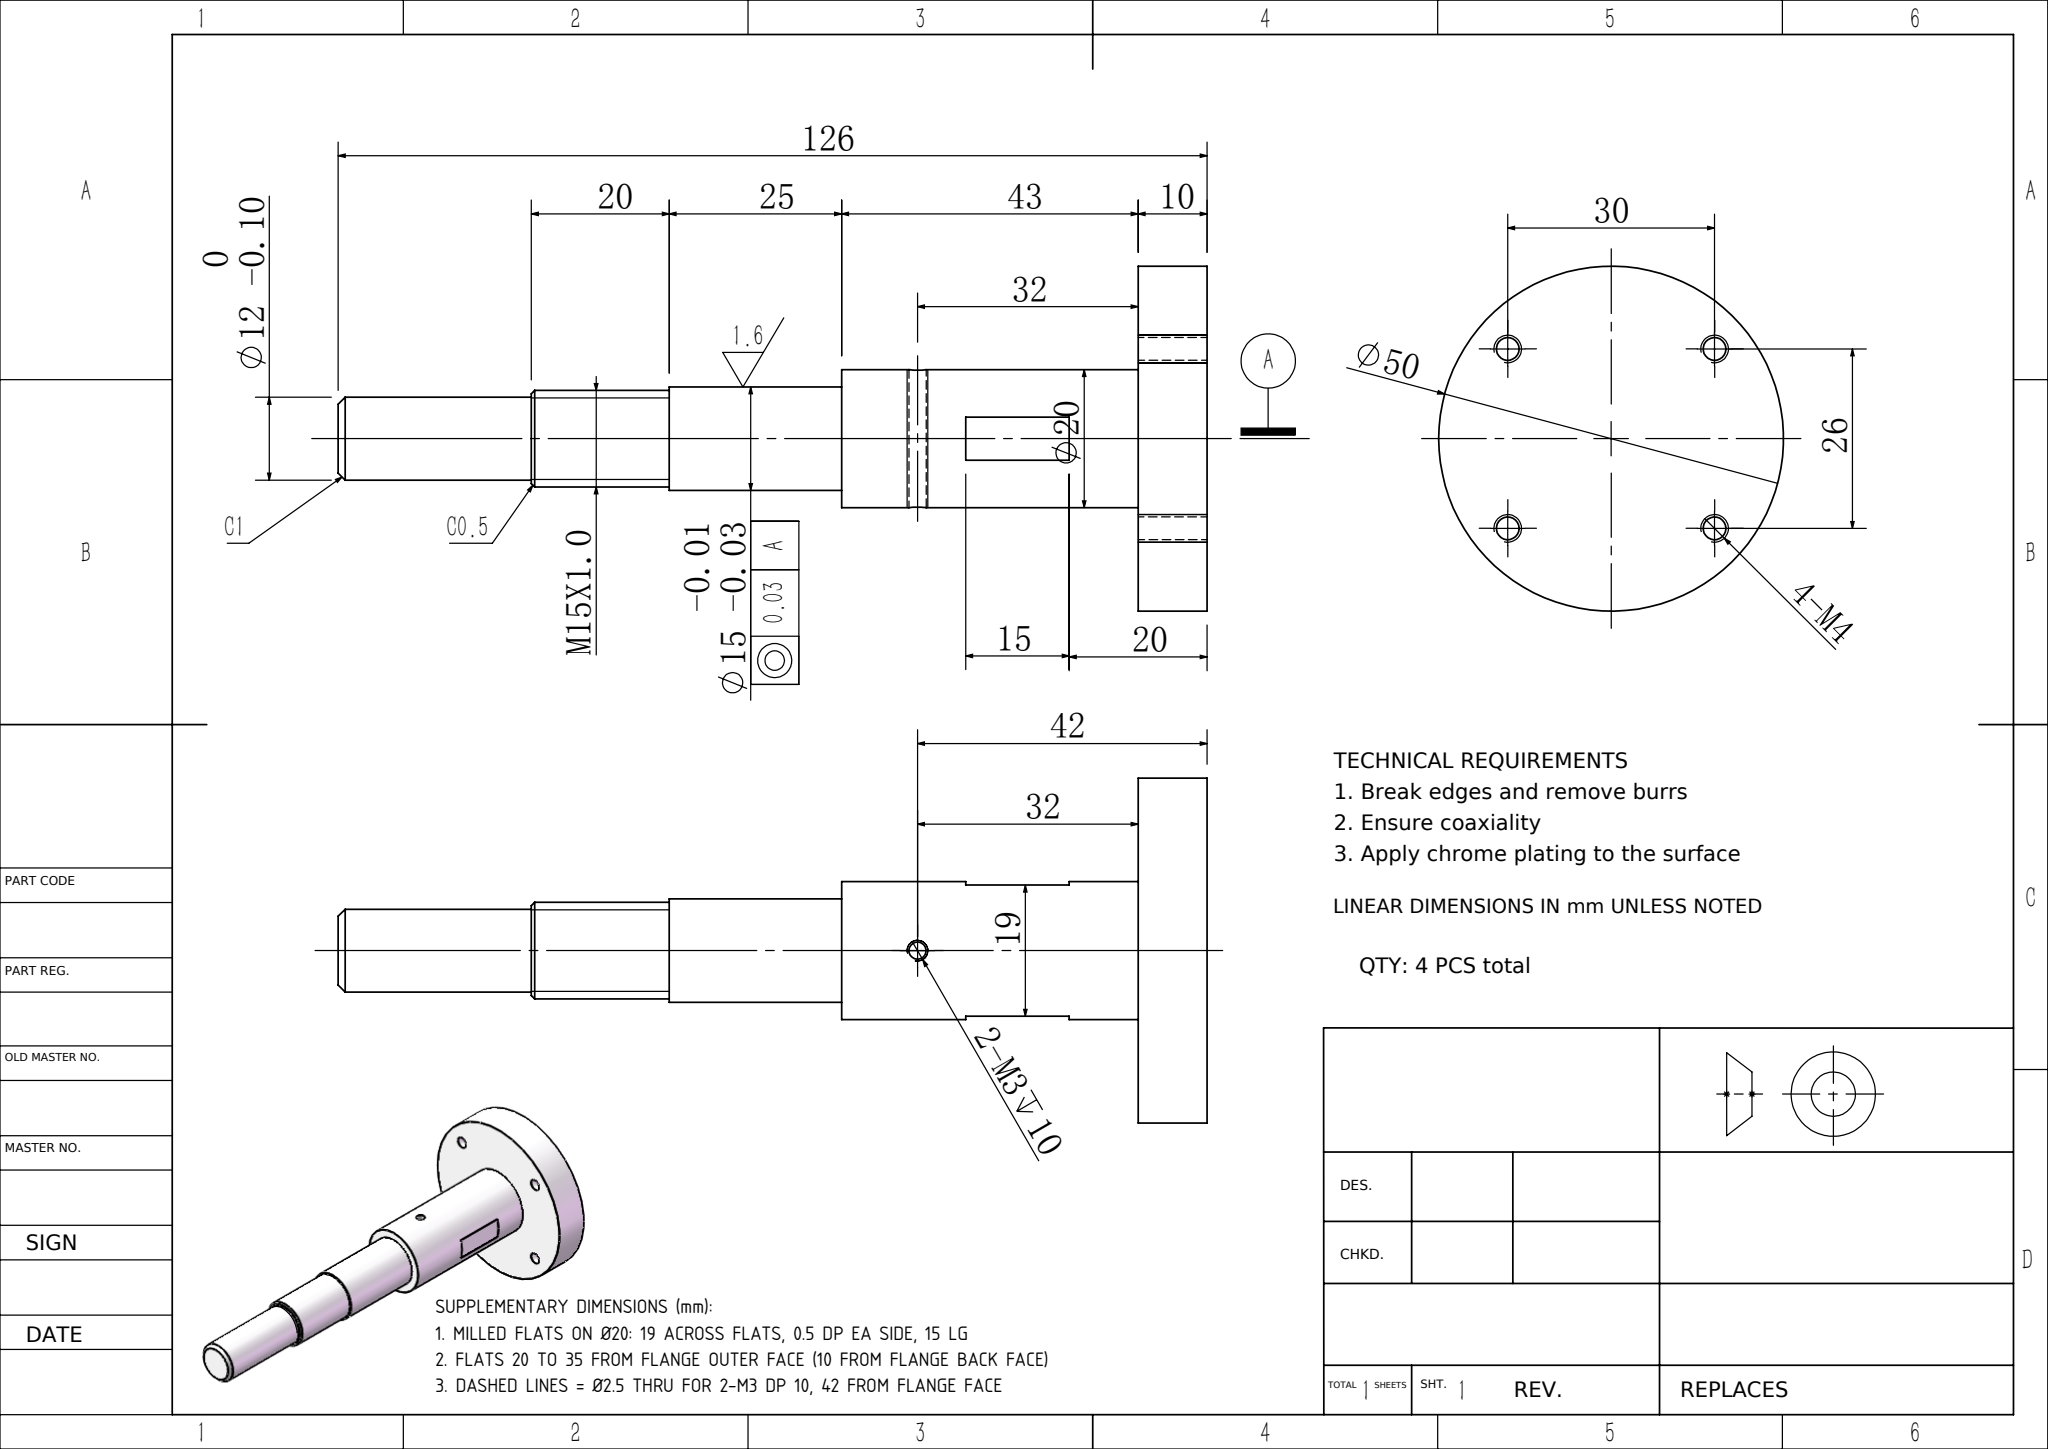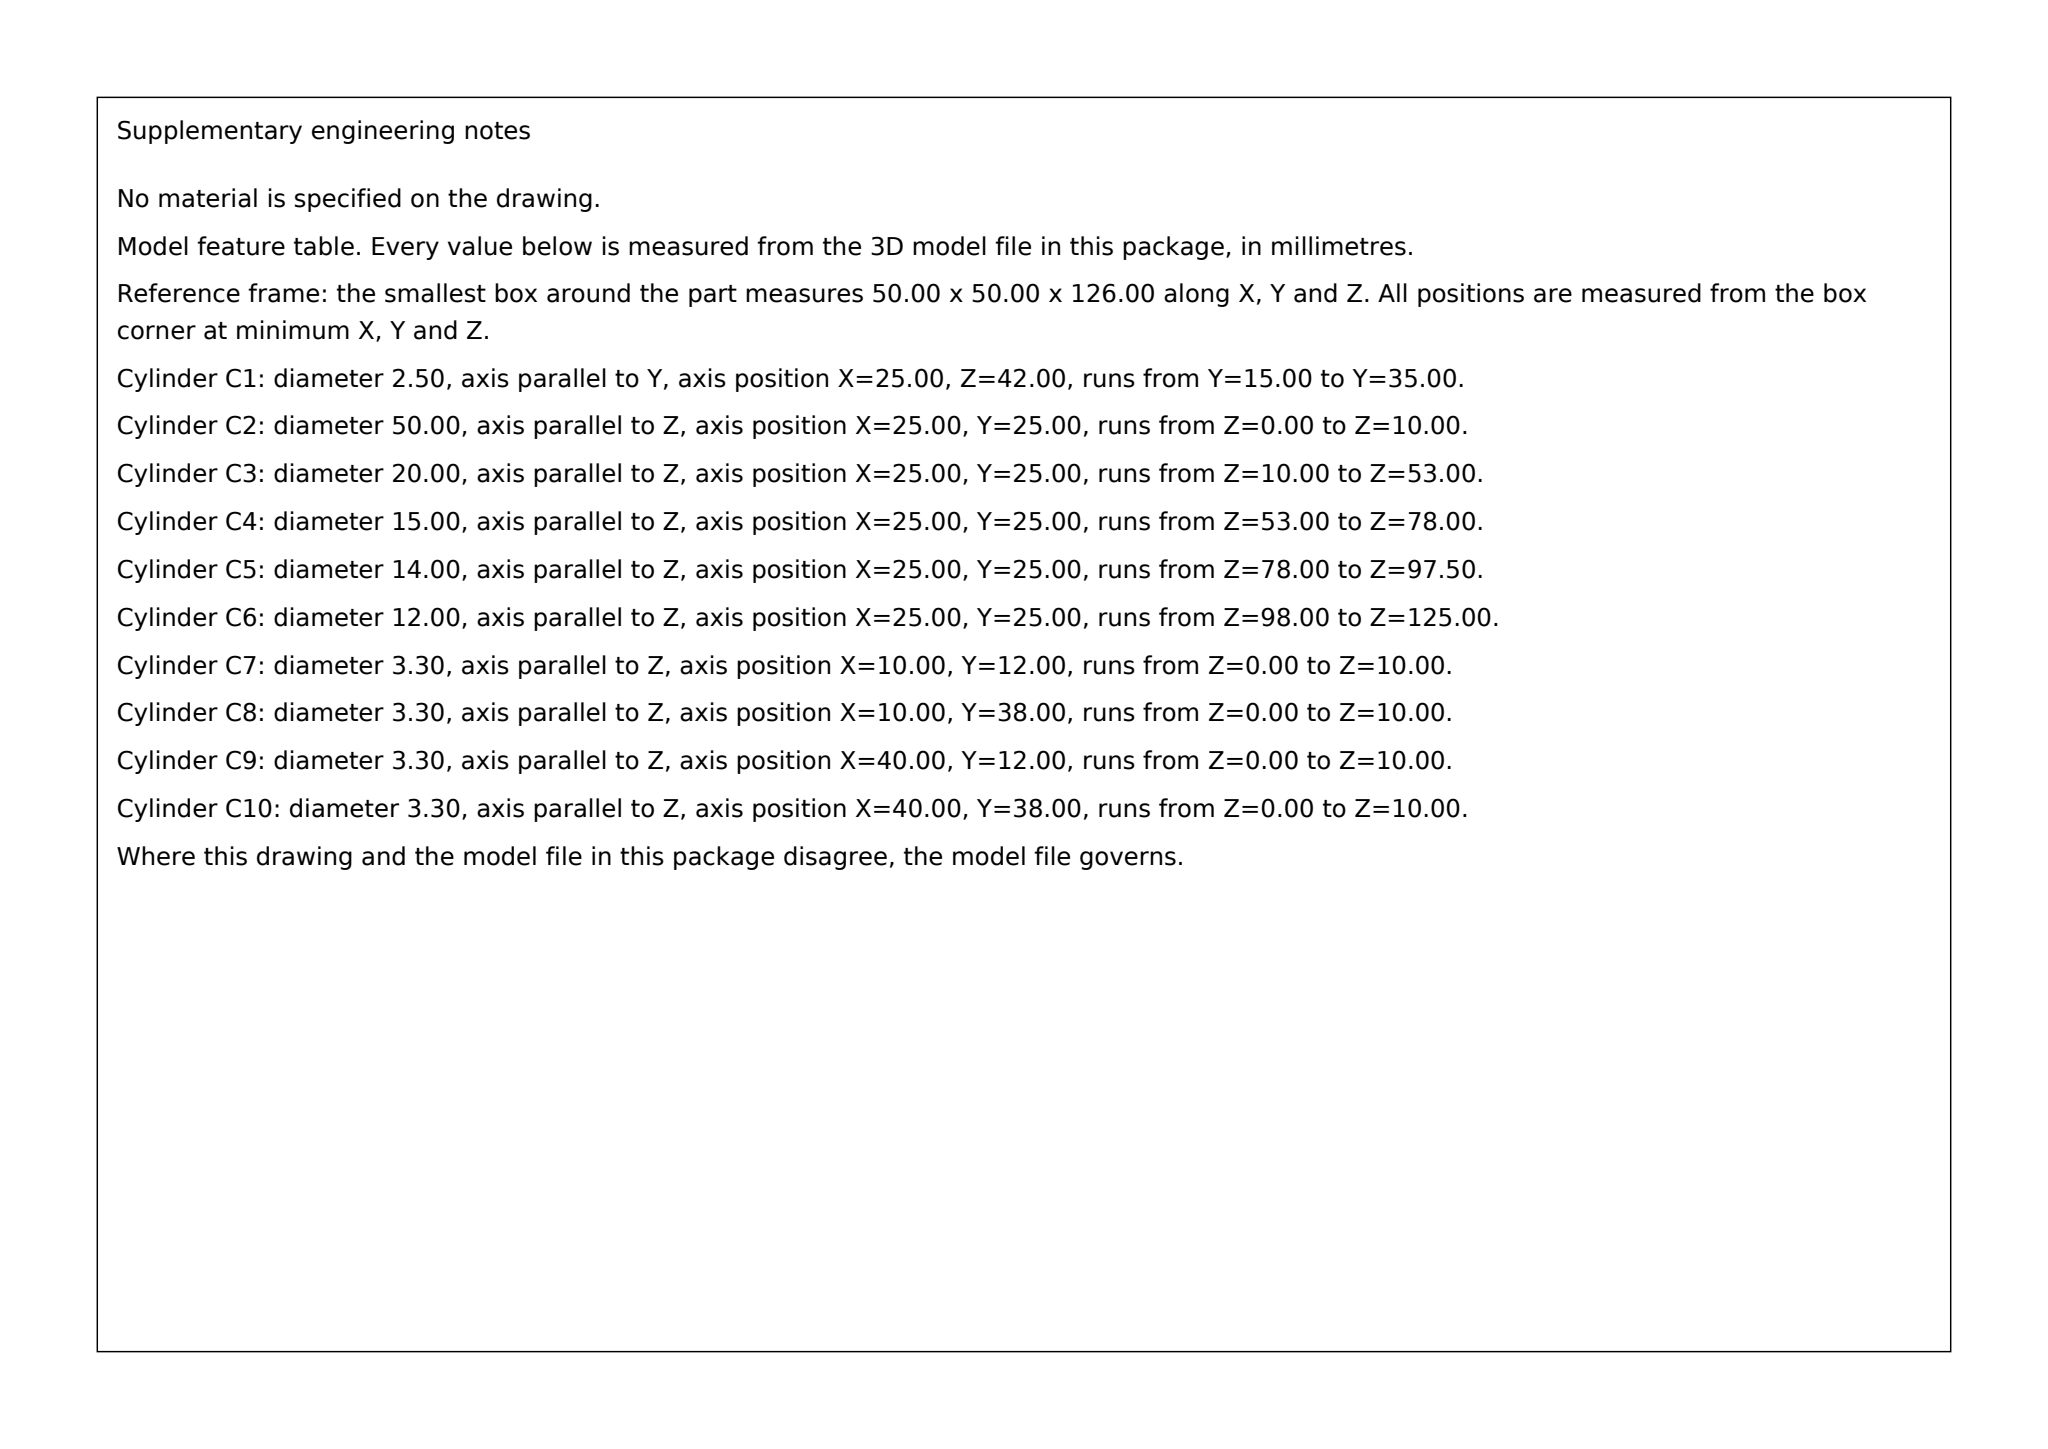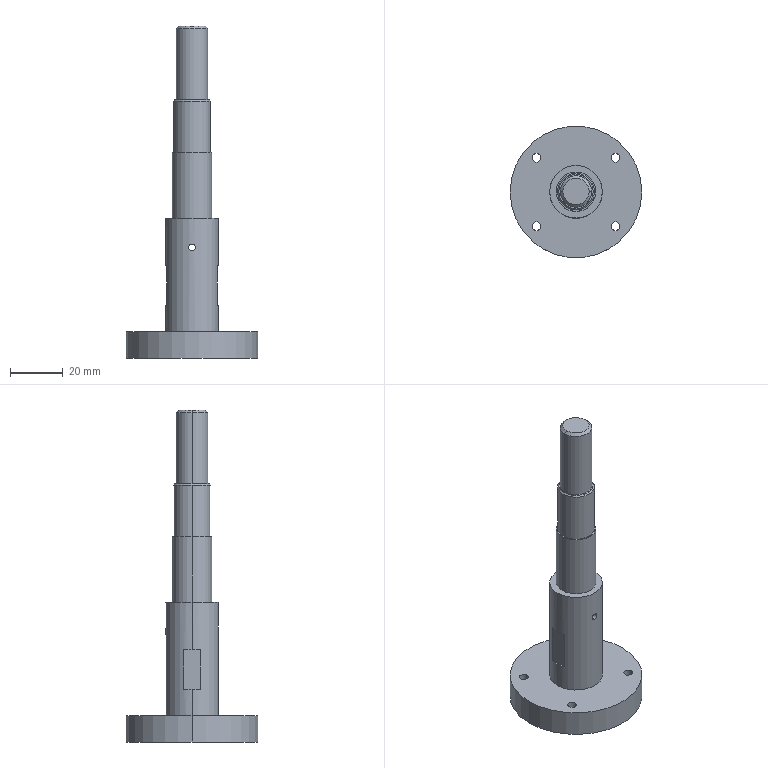Part | SolidWorks | mm | 1 solid | 36 faces | box 50 x 50 x 126 mm | volume 43281 mm3 | cylinder 20 | plane 12 | cone 4 | commonest cylinder face diameters 3.3 x8 2.5 x2 12 x2 14 x2 15 x2 50 x2 20 x2
build123d program:
from build123d import *

# Parameters (mm, degrees)
SKETCH1_R           = 25
BOSS_EXTRUDE1_DEPTH = 10
SKETCH2_R           = 10
BOSS_EXTRUDE2_DEPTH = 43
CUT_EXTRUDE1_START  = -18
SKETCH3_OUTSIDE_W   = 69.674
SKETCH3_OUTSIDE_H   = 69.674
SKETCH3_OUTSIDE_W_2 = 19
SKETCH3_OUTSIDE_H_2 = 33.791
CUT_EXTRUDE1_DEPTH  = 15
SKETCH4_R           = 1
CUT_EXTRUDE2_DEPTH  = 25
SKETCH5_R           = 7.5
BOSS_EXTRUDE3_DEPTH = 25
SKETCH6_R           = 7
BOSS_EXTRUDE4_DEPTH = 20
SKETCH7_R           = 6
BOSS_EXTRUDE5_DEPTH = 28
CHAMFER1_SIZE       = 1
CHAMFER2_SIZE       = 0.5
M4_TAPPED_HOLE1_D   = 3.3
SKETCH12_W          = 1.25
SKETCH12_H          = 25


with BuildPart() as part:
    # Sketch1 → Boss-Extrude1 (new body)
    with BuildSketch(Plane.XY):
        Circle(SKETCH1_R)
    extrude(amount=BOSS_EXTRUDE1_DEPTH)

    # Sketch2 → Boss-Extrude2 (add)
    with BuildSketch(Plane.XY.offset(10)):
        Circle(SKETCH2_R)
    extrude(amount=BOSS_EXTRUDE2_DEPTH)

    # Sketch3 outside → Cut-Extrude1 (cut)
    with BuildSketch(Plane.XY.offset(53).offset(CUT_EXTRUDE1_START)):
        Rectangle(SKETCH3_OUTSIDE_W, SKETCH3_OUTSIDE_H)
        Rectangle(SKETCH3_OUTSIDE_W_2, SKETCH3_OUTSIDE_H_2, mode=Mode.SUBTRACT)
    extrude(amount=-CUT_EXTRUDE1_DEPTH, mode=Mode.SUBTRACT)

    # Sketch4 → Cut-Extrude2 (cut, symmetric)
    with BuildSketch(Plane(origin=(0, 0, 0), x_dir=(1, 0, 0), z_dir=(0, 1, 0))):
        with Locations(Location((0, -42, 0), (0, 0, 270))):
            Circle(SKETCH4_R)
    extrude(amount=CUT_EXTRUDE2_DEPTH, both=True, mode=Mode.SUBTRACT)

    # Sketch5 → Boss-Extrude3 (add)
    with BuildSketch(Plane.XY.offset(53)):
        Circle(SKETCH5_R)
    extrude(amount=BOSS_EXTRUDE3_DEPTH)

    # Sketch6 → Boss-Extrude4 (add)
    with BuildSketch(Plane.XY.offset(78)):
        Circle(SKETCH6_R)
    extrude(amount=BOSS_EXTRUDE4_DEPTH)

    # Sketch7 → Boss-Extrude5 (add)
    with BuildSketch(Plane.XY.offset(98)):
        Circle(SKETCH7_R)
    extrude(amount=BOSS_EXTRUDE5_DEPTH)

    # Chamfer1
    chamfer1_edges = [part.edges().sort_by_distance(p)[0] for p in [
        (-6, 0, 126),
    ]]
    chamfer(chamfer1_edges, length=CHAMFER1_SIZE)

    # Chamfer2
    chamfer2_edges = [part.edges().sort_by_distance(p)[0] for p in [
        (-7, 0, 98),
    ]]
    chamfer(chamfer2_edges, length=CHAMFER2_SIZE)

    # M4 Tapped Hole1 (through all)
    with Locations(Plane(origin=(0, 0, 0), x_dir=(-1, 0, 0), z_dir=(0, 0, -1))):
        with Locations((-15, 13), (15, 13), (15, -13), (-15, -13)):
            Hole(M4_TAPPED_HOLE1_D / 2)

    # Sketch12 → M3 Tapped Hole1 (revolve, cut)
    with BuildSketch(Plane(origin=(0, 0, 42), x_dir=(0, 0, -1), z_dir=(1, 0, 0))):
        with Locations((0.625, 12.5)):
            Rectangle(SKETCH12_W, SKETCH12_H)
    m3_tapped_hole1 = revolve(axis=Axis((0, -6.35, 42), (0, 1, 0)), mode=Mode.SUBTRACT)

    # Mirror1: M3 Tapped Hole1 across plane
    add(m3_tapped_hole1.mirror(Plane.ZX), mode=Mode.SUBTRACT)


solid = part.part